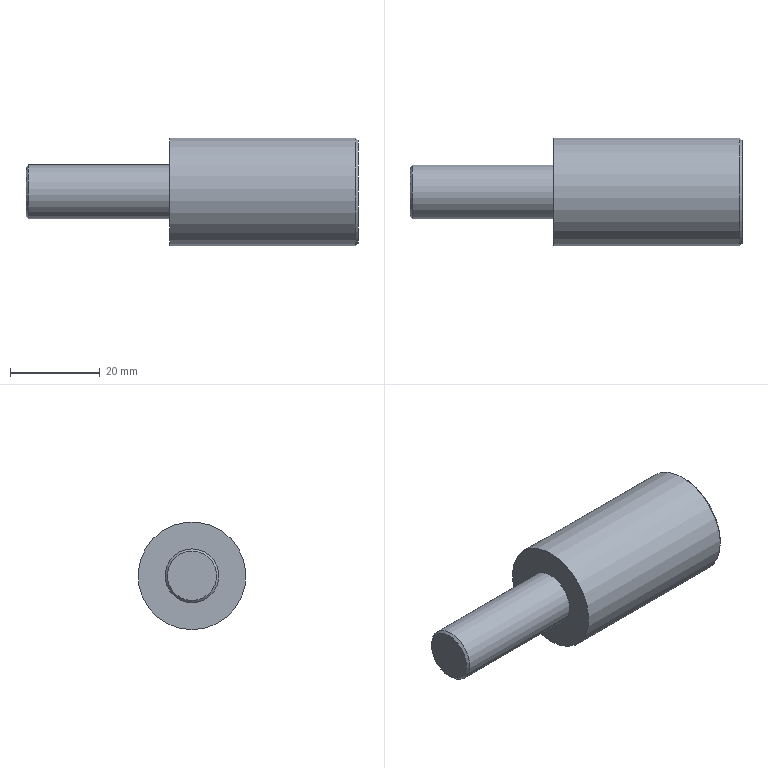Component | NX | CONNECTING_PIN | 1 solid | 7 faces | box 74 x 24 x 24 mm | volume 22606 mm3 | plane 3 | cylinder 2 | cone 2 | commonest cylinder face diameters 12 x1 24 x1
STEP:
#1=CARTESIAN_POINT('',(0.,0.,0.));
#2=DIRECTION('',(0.,0.,1.));
#3=DIRECTION('',(1.,0.,0.));
#4=AXIS2_PLACEMENT_3D('',#1,#2,#3);
#5=CARTESIAN_POINT('',(-16.,0.,193.));
#6=VERTEX_POINT('',#5);
#7=CARTESIAN_POINT('',(-16.,0.,187.5));
#8=DIRECTION('',(-1.,0.,0.));
#9=DIRECTION('',(0.,0.,1.));
#10=AXIS2_PLACEMENT_3D('',#7,#8,#9);
#11=CIRCLE('',#10,5.5);
#12=CARTESIAN_POINT('',(-16.,0.,187.5));
#13=DIRECTION('',(-1.,0.,0.));
#14=DIRECTION('',(0.,0.,1.));
#15=AXIS2_PLACEMENT_3D('',#12,#13,#14);
#16=PLANE('',#15);
#17=CARTESIAN_POINT('',(0.,0.));
#18=DIRECTION('',(1.,0.));
#19=AXIS2_PLACEMENT_2D('',#17,#18);
#20=CIRCLE('',#19,5.5);
#21=(GEOMETRIC_REPRESENTATION_CONTEXT(2)PARAMETRIC_REPRESENTATION_CONTEXT()REPRESENTATION_CONTEXT('',''));
#22=DEFINITIONAL_REPRESENTATION('',(#20),#21);
#23=PCURVE('',#16,#22);
#24=CARTESIAN_POINT('',(-15.5,0.,187.5));
#25=DIRECTION('',(1.,0.,0.));
#26=DIRECTION('',(0.,0.,-1.));
#27=AXIS2_PLACEMENT_3D('',#24,#25,#26);
#28=CONICAL_SURFACE('',#27,6.,0.7854);
#29=CARTESIAN_POINT('',(9.425,-0.5));
#30=DIRECTION('',(-1.,0.));
#31=VECTOR('',#30,1.);
#32=LINE('',#29,#31);
#33=(GEOMETRIC_REPRESENTATION_CONTEXT(2)PARAMETRIC_REPRESENTATION_CONTEXT()REPRESENTATION_CONTEXT('',''));
#34=DEFINITIONAL_REPRESENTATION('',(#32),#33);
#35=PCURVE('',#28,#34);
#36=SURFACE_CURVE('',#11,(#23,#35),.PCURVE_S1.);
#37=EDGE_CURVE('',#6,#6,#36,.T.);
#38=ORIENTED_EDGE('',*,*,#37,.T.);
#39=EDGE_LOOP('',(#38));
#40=FACE_BOUND('',#39,.T.);
#41=ADVANCED_FACE('',(#40),#16,.T.);
#42=CARTESIAN_POINT('',(-15.5,0.,193.5));
#43=VERTEX_POINT('',#42);
#44=CARTESIAN_POINT('',(-15.5,-0.,181.5));
#45=VERTEX_POINT('',#44);
#46=CARTESIAN_POINT('',(-15.5,0.,187.5));
#47=DIRECTION('',(1.,0.,0.));
#48=DIRECTION('',(0.,0.,1.));
#49=AXIS2_PLACEMENT_3D('',#46,#47,#48);
#50=CIRCLE('',#49,6.);
#51=CARTESIAN_POINT('',(-16.,0.,187.5));
#52=DIRECTION('',(1.,0.,0.));
#53=DIRECTION('',(0.,0.,-1.));
#54=AXIS2_PLACEMENT_3D('',#51,#52,#53);
#55=CYLINDRICAL_SURFACE('',#54,6.);
#56=CARTESIAN_POINT('',(3.142,0.5));
#57=DIRECTION('',(1.,0.));
#58=VECTOR('',#57,1.);
#59=LINE('',#56,#58);
#60=(GEOMETRIC_REPRESENTATION_CONTEXT(2)PARAMETRIC_REPRESENTATION_CONTEXT()REPRESENTATION_CONTEXT('',''));
#61=DEFINITIONAL_REPRESENTATION('',(#59),#60);
#62=PCURVE('',#55,#61);
#63=CARTESIAN_POINT('',(3.142,0.));
#64=DIRECTION('',(1.,0.));
#65=VECTOR('',#64,1.);
#66=LINE('',#63,#65);
#67=(GEOMETRIC_REPRESENTATION_CONTEXT(2)PARAMETRIC_REPRESENTATION_CONTEXT()REPRESENTATION_CONTEXT('',''));
#68=DEFINITIONAL_REPRESENTATION('',(#66),#67);
#69=PCURVE('',#28,#68);
#70=SURFACE_CURVE('',#50,(#62,#69),.PCURVE_S1.);
#71=EDGE_CURVE('',#43,#45,#70,.T.);
#72=ORIENTED_EDGE('',*,*,#71,.T.);
#73=CARTESIAN_POINT('',(16.,0.,181.5));
#74=VERTEX_POINT('',#73);
#75=CARTESIAN_POINT('',(-15.5,0.,181.5));
#76=CARTESIAN_POINT('',(16.,0.,181.5));
#77=B_SPLINE_CURVE_WITH_KNOTS('',1,(#75,#76),.UNSPECIFIED.,.F.,.F.,(2,2),(0.5,32.),.PIECEWISE_BEZIER_KNOTS.);
#78=CARTESIAN_POINT('',(6.283,0.));
#79=DIRECTION('',(0.,1.));
#80=VECTOR('',#79,1.);
#81=LINE('',#78,#80);
#82=(GEOMETRIC_REPRESENTATION_CONTEXT(2)PARAMETRIC_REPRESENTATION_CONTEXT()REPRESENTATION_CONTEXT('',''));
#83=DEFINITIONAL_REPRESENTATION('',(#81),#82);
#84=PCURVE('',#55,#83);
#85=CARTESIAN_POINT('',(0.,0.));
#86=DIRECTION('',(0.,1.));
#87=VECTOR('',#86,1.);
#88=LINE('',#85,#87);
#89=(GEOMETRIC_REPRESENTATION_CONTEXT(2)PARAMETRIC_REPRESENTATION_CONTEXT()REPRESENTATION_CONTEXT('',''));
#90=DEFINITIONAL_REPRESENTATION('',(#88),#89);
#91=PCURVE('',#55,#90);
#92=SEAM_CURVE('',#77,(#84,#91),.PCURVE_S1.);
#93=EDGE_CURVE('',#45,#74,#92,.T.);
#94=ORIENTED_EDGE('',*,*,#93,.T.);
#95=CARTESIAN_POINT('',(16.,0.,187.5));
#96=DIRECTION('',(-1.,0.,0.));
#97=DIRECTION('',(0.,0.,-1.));
#98=AXIS2_PLACEMENT_3D('',#95,#96,#97);
#99=CIRCLE('',#98,6.);
#100=CARTESIAN_POINT('',(6.283,32.));
#101=DIRECTION('',(-1.,0.));
#102=VECTOR('',#101,1.);
#103=LINE('',#100,#102);
#104=(GEOMETRIC_REPRESENTATION_CONTEXT(2)PARAMETRIC_REPRESENTATION_CONTEXT()REPRESENTATION_CONTEXT('',''));
#105=DEFINITIONAL_REPRESENTATION('',(#103),#104);
#106=PCURVE('',#55,#105);
#107=CARTESIAN_POINT('',(16.,-0.,187.5));
#108=DIRECTION('',(-1.,0.,0.));
#109=DIRECTION('',(0.,0.,1.));
#110=AXIS2_PLACEMENT_3D('',#107,#108,#109);
#111=PLANE('',#110);
#112=CARTESIAN_POINT('',(0.,0.));
#113=DIRECTION('',(-1.,0.));
#114=AXIS2_PLACEMENT_2D('',#112,#113);
#115=CIRCLE('',#114,6.);
#116=(GEOMETRIC_REPRESENTATION_CONTEXT(2)PARAMETRIC_REPRESENTATION_CONTEXT()REPRESENTATION_CONTEXT('',''));
#117=DEFINITIONAL_REPRESENTATION('',(#115),#116);
#118=PCURVE('',#111,#117);
#119=SURFACE_CURVE('',#99,(#106,#118),.PCURVE_S1.);
#120=EDGE_CURVE('',#74,#74,#119,.T.);
#121=ORIENTED_EDGE('',*,*,#120,.T.);
#122=ORIENTED_EDGE('',*,*,#93,.F.);
#123=CARTESIAN_POINT('',(-15.5,0.,187.5));
#124=DIRECTION('',(1.,0.,0.));
#125=DIRECTION('',(0.,0.,1.));
#126=AXIS2_PLACEMENT_3D('',#123,#124,#125);
#127=CIRCLE('',#126,6.);
#128=CARTESIAN_POINT('',(-3.142,0.5));
#129=DIRECTION('',(1.,0.));
#130=VECTOR('',#129,1.);
#131=LINE('',#128,#130);
#132=(GEOMETRIC_REPRESENTATION_CONTEXT(2)PARAMETRIC_REPRESENTATION_CONTEXT()REPRESENTATION_CONTEXT('',''));
#133=DEFINITIONAL_REPRESENTATION('',(#131),#132);
#134=PCURVE('',#55,#133);
#135=CARTESIAN_POINT('',(3.142,0.));
#136=DIRECTION('',(1.,0.));
#137=VECTOR('',#136,1.);
#138=LINE('',#135,#137);
#139=(GEOMETRIC_REPRESENTATION_CONTEXT(2)PARAMETRIC_REPRESENTATION_CONTEXT()REPRESENTATION_CONTEXT('',''));
#140=DEFINITIONAL_REPRESENTATION('',(#138),#139);
#141=PCURVE('',#28,#140);
#142=SURFACE_CURVE('',#127,(#134,#141),.PCURVE_S1.);
#143=EDGE_CURVE('',#45,#43,#142,.T.);
#144=ORIENTED_EDGE('',*,*,#143,.T.);
#145=EDGE_LOOP('',(#72,#94,#121,#122,#144));
#146=FACE_BOUND('',#145,.T.);
#147=ADVANCED_FACE('',(#146),#55,.T.);
#148=CARTESIAN_POINT('',(58.,-0.,176.));
#149=VERTEX_POINT('',#148);
#150=CARTESIAN_POINT('',(58.,-0.,187.5));
#151=DIRECTION('',(1.,0.,0.));
#152=DIRECTION('',(0.,0.,-1.));
#153=AXIS2_PLACEMENT_3D('',#150,#151,#152);
#154=CIRCLE('',#153,11.5);
#155=CARTESIAN_POINT('',(58.,-0.,187.5));
#156=DIRECTION('',(1.,0.,0.));
#157=DIRECTION('',(0.,0.,-1.));
#158=AXIS2_PLACEMENT_3D('',#155,#156,#157);
#159=PLANE('',#158);
#160=CARTESIAN_POINT('',(0.,0.));
#161=DIRECTION('',(1.,0.));
#162=AXIS2_PLACEMENT_2D('',#160,#161);
#163=CIRCLE('',#162,11.5);
#164=(GEOMETRIC_REPRESENTATION_CONTEXT(2)PARAMETRIC_REPRESENTATION_CONTEXT()REPRESENTATION_CONTEXT('',''));
#165=DEFINITIONAL_REPRESENTATION('',(#163),#164);
#166=PCURVE('',#159,#165);
#167=CARTESIAN_POINT('',(58.,-0.,187.5));
#168=DIRECTION('',(-1.,0.,0.));
#169=DIRECTION('',(0.,0.,1.));
#170=AXIS2_PLACEMENT_3D('',#167,#168,#169);
#171=CONICAL_SURFACE('',#170,11.5,0.7854);
#172=CARTESIAN_POINT('',(9.425,0.));
#173=DIRECTION('',(-1.,0.));
#174=VECTOR('',#173,1.);
#175=LINE('',#172,#174);
#176=(GEOMETRIC_REPRESENTATION_CONTEXT(2)PARAMETRIC_REPRESENTATION_CONTEXT()REPRESENTATION_CONTEXT('',''));
#177=DEFINITIONAL_REPRESENTATION('',(#175),#176);
#178=PCURVE('',#171,#177);
#179=SURFACE_CURVE('',#154,(#166,#178),.PCURVE_S1.);
#180=EDGE_CURVE('',#149,#149,#179,.T.);
#181=ORIENTED_EDGE('',*,*,#180,.T.);
#182=EDGE_LOOP('',(#181));
#183=FACE_BOUND('',#182,.T.);
#184=ADVANCED_FACE('',(#183),#159,.T.);
#185=ORIENTED_EDGE('',*,*,#120,.F.);
#186=EDGE_LOOP('',(#185));
#187=FACE_BOUND('',#186,.T.);
#188=CARTESIAN_POINT('',(16.,-0.,175.5));
#189=VERTEX_POINT('',#188);
#190=CARTESIAN_POINT('',(16.,-0.,187.5));
#191=DIRECTION('',(1.,0.,0.));
#192=DIRECTION('',(0.,0.,-1.));
#193=AXIS2_PLACEMENT_3D('',#190,#191,#192);
#194=CIRCLE('',#193,12.);
#195=CARTESIAN_POINT('',(-12.,0.));
#196=CARTESIAN_POINT('',(-12.,20.785));
#197=CARTESIAN_POINT('',(6.,10.392));
#198=CARTESIAN_POINT('',(24.,0.));
#199=CARTESIAN_POINT('',(6.,-10.392));
#200=CARTESIAN_POINT('',(-12.,-20.785));
#201=CARTESIAN_POINT('',(-12.,0.));
#202=(BOUNDED_CURVE()B_SPLINE_CURVE(2,(#195,#196,#197,#198,#199,#200,#201),.UNSPECIFIED.,.T.,.F.)B_SPLINE_CURVE_WITH_KNOTS((1,2,2,2,2,1),(-2.094,0.,2.094,4.189,6.283,8.378),.UNSPECIFIED.)CURVE()GEOMETRIC_REPRESENTATION_ITEM()RATIONAL_B_SPLINE_CURVE((1.,0.5,1.,0.5,1.,0.5,1.))REPRESENTATION_ITEM(''));
#203=(GEOMETRIC_REPRESENTATION_CONTEXT(2)PARAMETRIC_REPRESENTATION_CONTEXT()REPRESENTATION_CONTEXT('',''));
#204=DEFINITIONAL_REPRESENTATION('',(#202),#203);
#205=PCURVE('',#111,#204);
#206=CARTESIAN_POINT('',(16.,-0.,187.5));
#207=DIRECTION('',(1.,0.,0.));
#208=DIRECTION('',(0.,0.,-1.));
#209=AXIS2_PLACEMENT_3D('',#206,#207,#208);
#210=CYLINDRICAL_SURFACE('',#209,12.);
#211=CARTESIAN_POINT('',(0.,0.));
#212=DIRECTION('',(1.,0.));
#213=VECTOR('',#212,1.);
#214=LINE('',#211,#213);
#215=(GEOMETRIC_REPRESENTATION_CONTEXT(2)PARAMETRIC_REPRESENTATION_CONTEXT()REPRESENTATION_CONTEXT('',''));
#216=DEFINITIONAL_REPRESENTATION('',(#214),#215);
#217=PCURVE('',#210,#216);
#218=SURFACE_CURVE('',#194,(#205,#217),.PCURVE_S1.);
#219=EDGE_CURVE('',#189,#189,#218,.T.);
#220=ORIENTED_EDGE('',*,*,#219,.F.);
#221=EDGE_LOOP('',(#220));
#222=FACE_BOUND('',#221,.T.);
#223=ADVANCED_FACE('',(#187,#222),#111,.T.);
#224=CARTESIAN_POINT('',(57.5,-0.,175.5));
#225=VERTEX_POINT('',#224);
#226=CARTESIAN_POINT('',(57.5,-0.,187.5));
#227=DIRECTION('',(-1.,0.,0.));
#228=DIRECTION('',(0.,0.,-1.));
#229=AXIS2_PLACEMENT_3D('',#226,#227,#228);
#230=CIRCLE('',#229,12.);
#231=CARTESIAN_POINT('',(6.283,41.5));
#232=DIRECTION('',(-1.,0.));
#233=VECTOR('',#232,1.);
#234=LINE('',#231,#233);
#235=(GEOMETRIC_REPRESENTATION_CONTEXT(2)PARAMETRIC_REPRESENTATION_CONTEXT()REPRESENTATION_CONTEXT('',''));
#236=DEFINITIONAL_REPRESENTATION('',(#234),#235);
#237=PCURVE('',#210,#236);
#238=CARTESIAN_POINT('',(3.142,0.5));
#239=DIRECTION('',(1.,0.));
#240=VECTOR('',#239,1.);
#241=LINE('',#238,#240);
#242=(GEOMETRIC_REPRESENTATION_CONTEXT(2)PARAMETRIC_REPRESENTATION_CONTEXT()REPRESENTATION_CONTEXT('',''));
#243=DEFINITIONAL_REPRESENTATION('',(#241),#242);
#244=PCURVE('',#171,#243);
#245=SURFACE_CURVE('',#230,(#237,#244),.PCURVE_S1.);
#246=EDGE_CURVE('',#225,#225,#245,.T.);
#247=ORIENTED_EDGE('',*,*,#246,.T.);
#248=CARTESIAN_POINT('',(16.,-0.,175.5));
#249=CARTESIAN_POINT('',(57.5,-0.,175.5));
#250=B_SPLINE_CURVE_WITH_KNOTS('',1,(#248,#249),.UNSPECIFIED.,.F.,.F.,(2,2),(0.,41.5),.PIECEWISE_BEZIER_KNOTS.);
#251=CARTESIAN_POINT('',(0.,0.));
#252=DIRECTION('',(0.,1.));
#253=VECTOR('',#252,1.);
#254=LINE('',#251,#253);
#255=(GEOMETRIC_REPRESENTATION_CONTEXT(2)PARAMETRIC_REPRESENTATION_CONTEXT()REPRESENTATION_CONTEXT('',''));
#256=DEFINITIONAL_REPRESENTATION('',(#254),#255);
#257=PCURVE('',#210,#256);
#258=CARTESIAN_POINT('',(6.283,0.));
#259=DIRECTION('',(0.,1.));
#260=VECTOR('',#259,1.);
#261=LINE('',#258,#260);
#262=(GEOMETRIC_REPRESENTATION_CONTEXT(2)PARAMETRIC_REPRESENTATION_CONTEXT()REPRESENTATION_CONTEXT('',''));
#263=DEFINITIONAL_REPRESENTATION('',(#261),#262);
#264=PCURVE('',#210,#263);
#265=SEAM_CURVE('',#250,(#257,#264),.PCURVE_S1.);
#266=EDGE_CURVE('',#189,#225,#265,.T.);
#267=ORIENTED_EDGE('',*,*,#266,.F.);
#268=ORIENTED_EDGE('',*,*,#219,.T.);
#269=ORIENTED_EDGE('',*,*,#266,.T.);
#270=EDGE_LOOP('',(#247,#267,#268,#269));
#271=FACE_BOUND('',#270,.T.);
#272=ADVANCED_FACE('',(#271),#210,.T.);
#273=ORIENTED_EDGE('',*,*,#246,.F.);
#274=CARTESIAN_POINT('',(58.,0.,176.));
#275=CARTESIAN_POINT('',(57.5,0.,175.5));
#276=B_SPLINE_CURVE_WITH_KNOTS('',1,(#274,#275),.UNSPECIFIED.,.F.,.F.,(2,2),(0.,0.7071),.PIECEWISE_BEZIER_KNOTS.);
#277=CARTESIAN_POINT('',(3.142,0.));
#278=DIRECTION('',(0.,1.));
#279=VECTOR('',#278,1.);
#280=LINE('',#277,#279);
#281=(GEOMETRIC_REPRESENTATION_CONTEXT(2)PARAMETRIC_REPRESENTATION_CONTEXT()REPRESENTATION_CONTEXT('',''));
#282=DEFINITIONAL_REPRESENTATION('',(#280),#281);
#283=PCURVE('',#171,#282);
#284=CARTESIAN_POINT('',(9.425,0.));
#285=DIRECTION('',(0.,1.));
#286=VECTOR('',#285,1.);
#287=LINE('',#284,#286);
#288=(GEOMETRIC_REPRESENTATION_CONTEXT(2)PARAMETRIC_REPRESENTATION_CONTEXT()REPRESENTATION_CONTEXT('',''));
#289=DEFINITIONAL_REPRESENTATION('',(#287),#288);
#290=PCURVE('',#171,#289);
#291=SEAM_CURVE('',#276,(#283,#290),.PCURVE_S1.);
#292=EDGE_CURVE('',#149,#225,#291,.T.);
#293=ORIENTED_EDGE('',*,*,#292,.F.);
#294=ORIENTED_EDGE('',*,*,#180,.F.);
#295=ORIENTED_EDGE('',*,*,#292,.T.);
#296=EDGE_LOOP('',(#273,#293,#294,#295));
#297=FACE_BOUND('',#296,.T.);
#298=ADVANCED_FACE('',(#297),#171,.T.);
#299=ORIENTED_EDGE('',*,*,#37,.F.);
#300=CARTESIAN_POINT('',(-16.,0.,193.));
#301=CARTESIAN_POINT('',(-15.5,0.,193.5));
#302=B_SPLINE_CURVE_WITH_KNOTS('',1,(#300,#301),.UNSPECIFIED.,.F.,.F.,(2,2),(-0.7071,0.),.PIECEWISE_BEZIER_KNOTS.);
#303=CARTESIAN_POINT('',(9.425,0.));
#304=DIRECTION('',(0.,1.));
#305=VECTOR('',#304,1.);
#306=LINE('',#303,#305);
#307=(GEOMETRIC_REPRESENTATION_CONTEXT(2)PARAMETRIC_REPRESENTATION_CONTEXT()REPRESENTATION_CONTEXT('',''));
#308=DEFINITIONAL_REPRESENTATION('',(#306),#307);
#309=PCURVE('',#28,#308);
#310=CARTESIAN_POINT('',(3.142,0.));
#311=DIRECTION('',(0.,1.));
#312=VECTOR('',#311,1.);
#313=LINE('',#310,#312);
#314=(GEOMETRIC_REPRESENTATION_CONTEXT(2)PARAMETRIC_REPRESENTATION_CONTEXT()REPRESENTATION_CONTEXT('',''));
#315=DEFINITIONAL_REPRESENTATION('',(#313),#314);
#316=PCURVE('',#28,#315);
#317=SEAM_CURVE('',#302,(#309,#316),.PCURVE_S1.);
#318=EDGE_CURVE('',#6,#43,#317,.T.);
#319=ORIENTED_EDGE('',*,*,#318,.T.);
#320=ORIENTED_EDGE('',*,*,#143,.F.);
#321=ORIENTED_EDGE('',*,*,#71,.F.);
#322=ORIENTED_EDGE('',*,*,#318,.F.);
#323=EDGE_LOOP('',(#299,#319,#320,#321,#322));
#324=FACE_BOUND('',#323,.T.);
#325=ADVANCED_FACE('',(#324),#28,.T.);
#326=CLOSED_SHELL('',(#41,#147,#184,#223,#272,#298,#325));
#327=MANIFOLD_SOLID_BREP('',#326);
#328=(LENGTH_UNIT()NAMED_UNIT(*)SI_UNIT(.MILLI.,.METRE.));
#329=UNCERTAINTY_MEASURE_WITH_UNIT(LENGTH_MEASURE(0.00001),#328,'','');
#330=(NAMED_UNIT(*)PLANE_ANGLE_UNIT()SI_UNIT($,.RADIAN.));
#331=(NAMED_UNIT(*)SI_UNIT($,.STERADIAN.)SOLID_ANGLE_UNIT());
#332=(GEOMETRIC_REPRESENTATION_CONTEXT(3)GLOBAL_UNCERTAINTY_ASSIGNED_CONTEXT((#329))GLOBAL_UNIT_ASSIGNED_CONTEXT((#328,#330,#331))REPRESENTATION_CONTEXT('',''));
#333=ADVANCED_BREP_SHAPE_REPRESENTATION('',(#4,#327),#332);